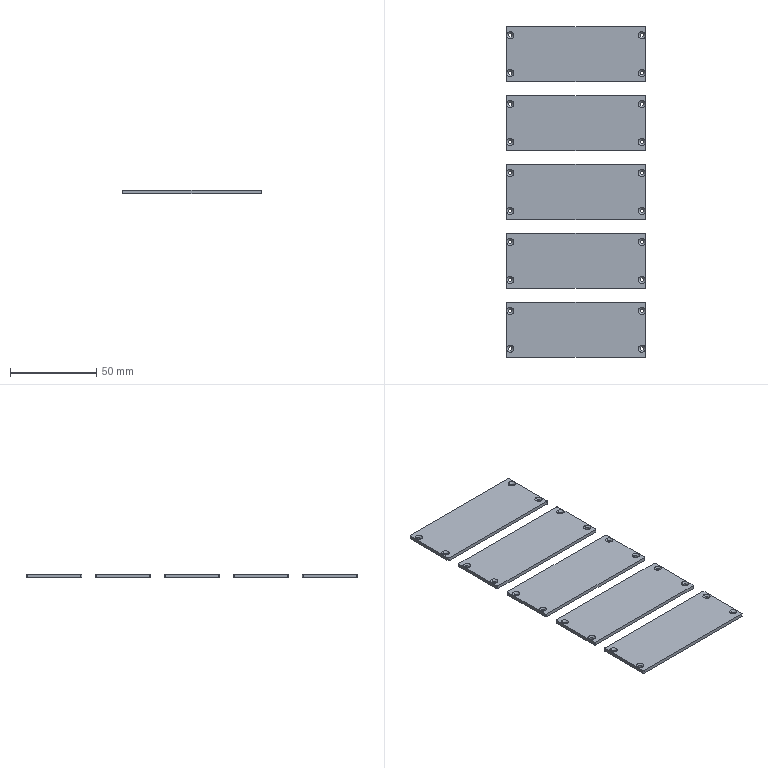CAM job | Mastercam | mm | 4 operations | part box 81.2 x 192 x 2
1. Contour (Ramp) | 3 - 3 平铣刀
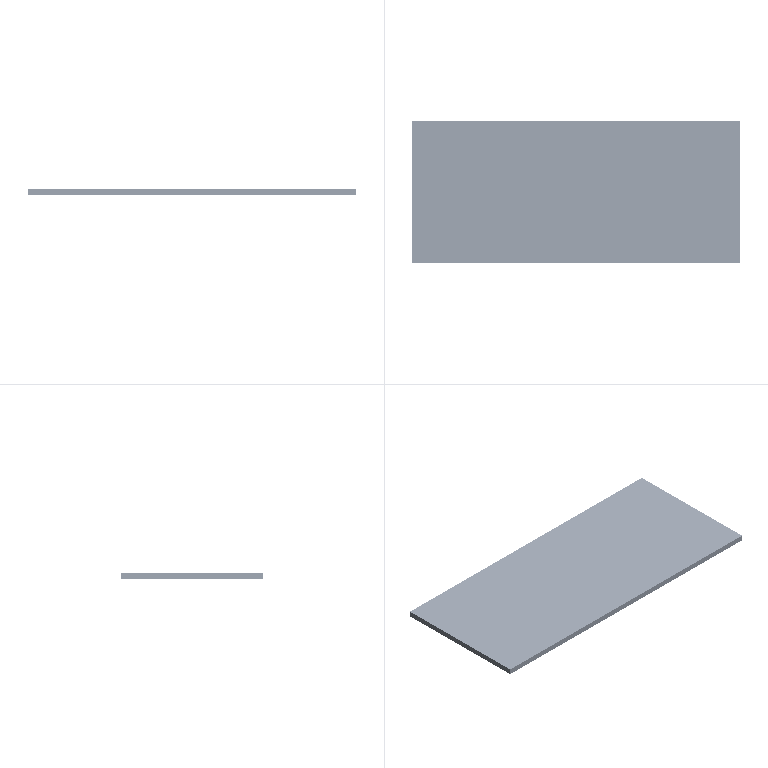2. Drill/Counterbore | 7 - 4 倒角刀
3. Contour (2D chamfer) | 7 - 4 倒角刀
4. Contour (2D) | 2 - 2 平铣刀